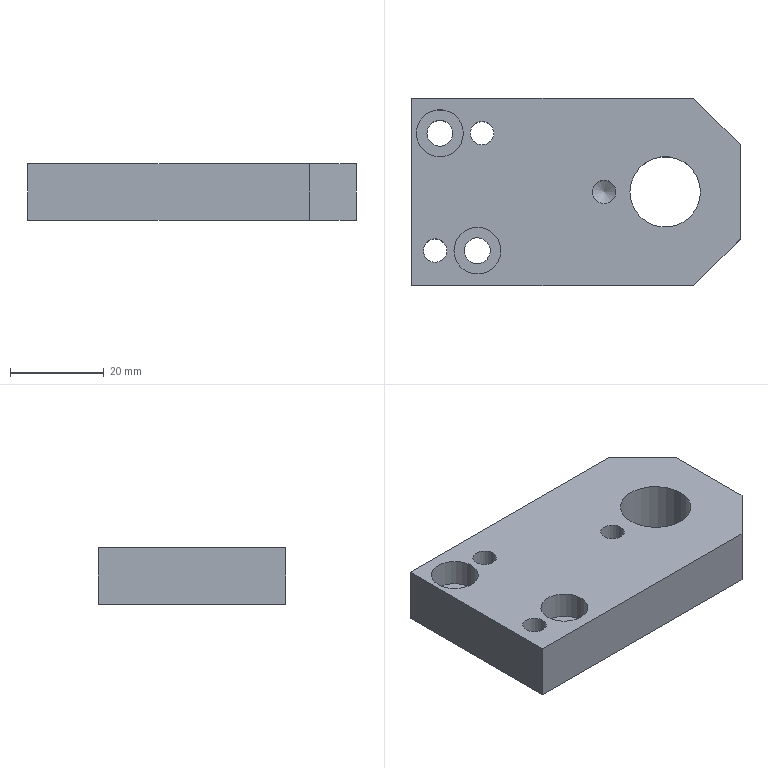Component | NX | DRILL_TEMPLATE | 1 solid | 19 faces | volume 28396 mm3 | plane 10 | cylinder 8 | cone 1 | commonest cylinder face diameters 5 x3 5.5 x2 10 x2 15 x1